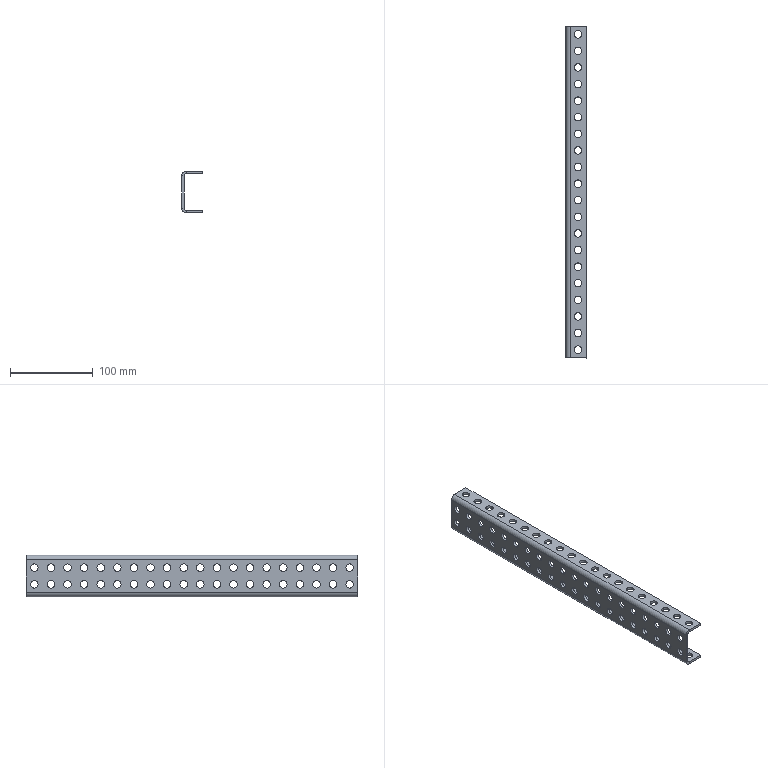Component | SolidWorks | MiddleColumnF2-01-1 | 1 solid | 182 faces | volume 93412 mm3 | cylinder 164 | plane 18 | commonest cylinder face diameters 9 x160 11 x2 5 x2